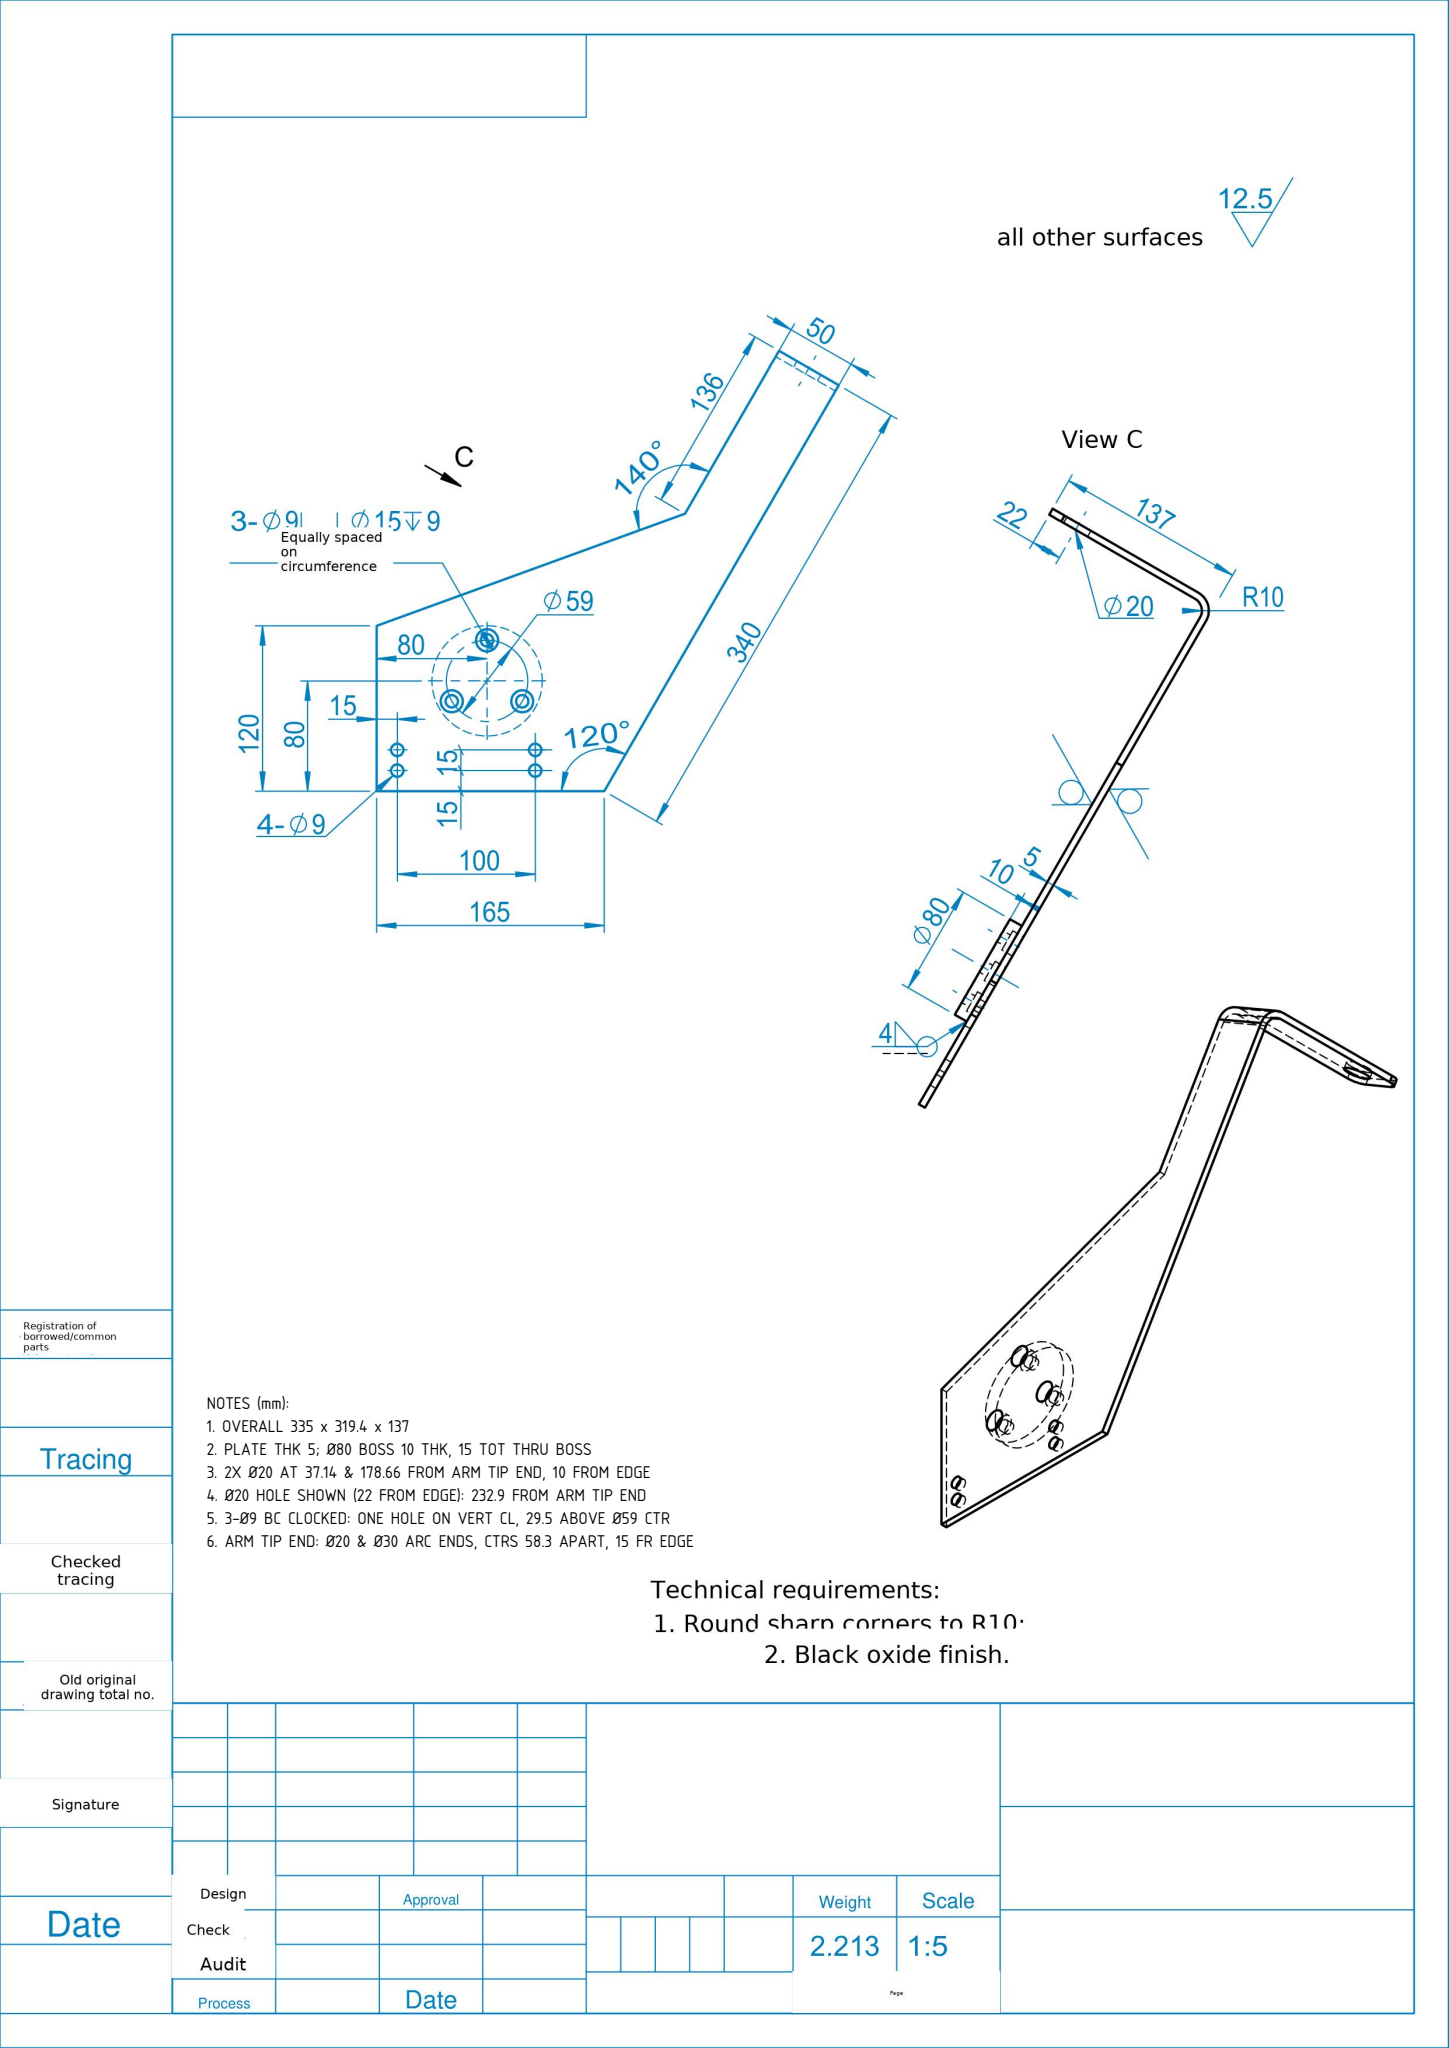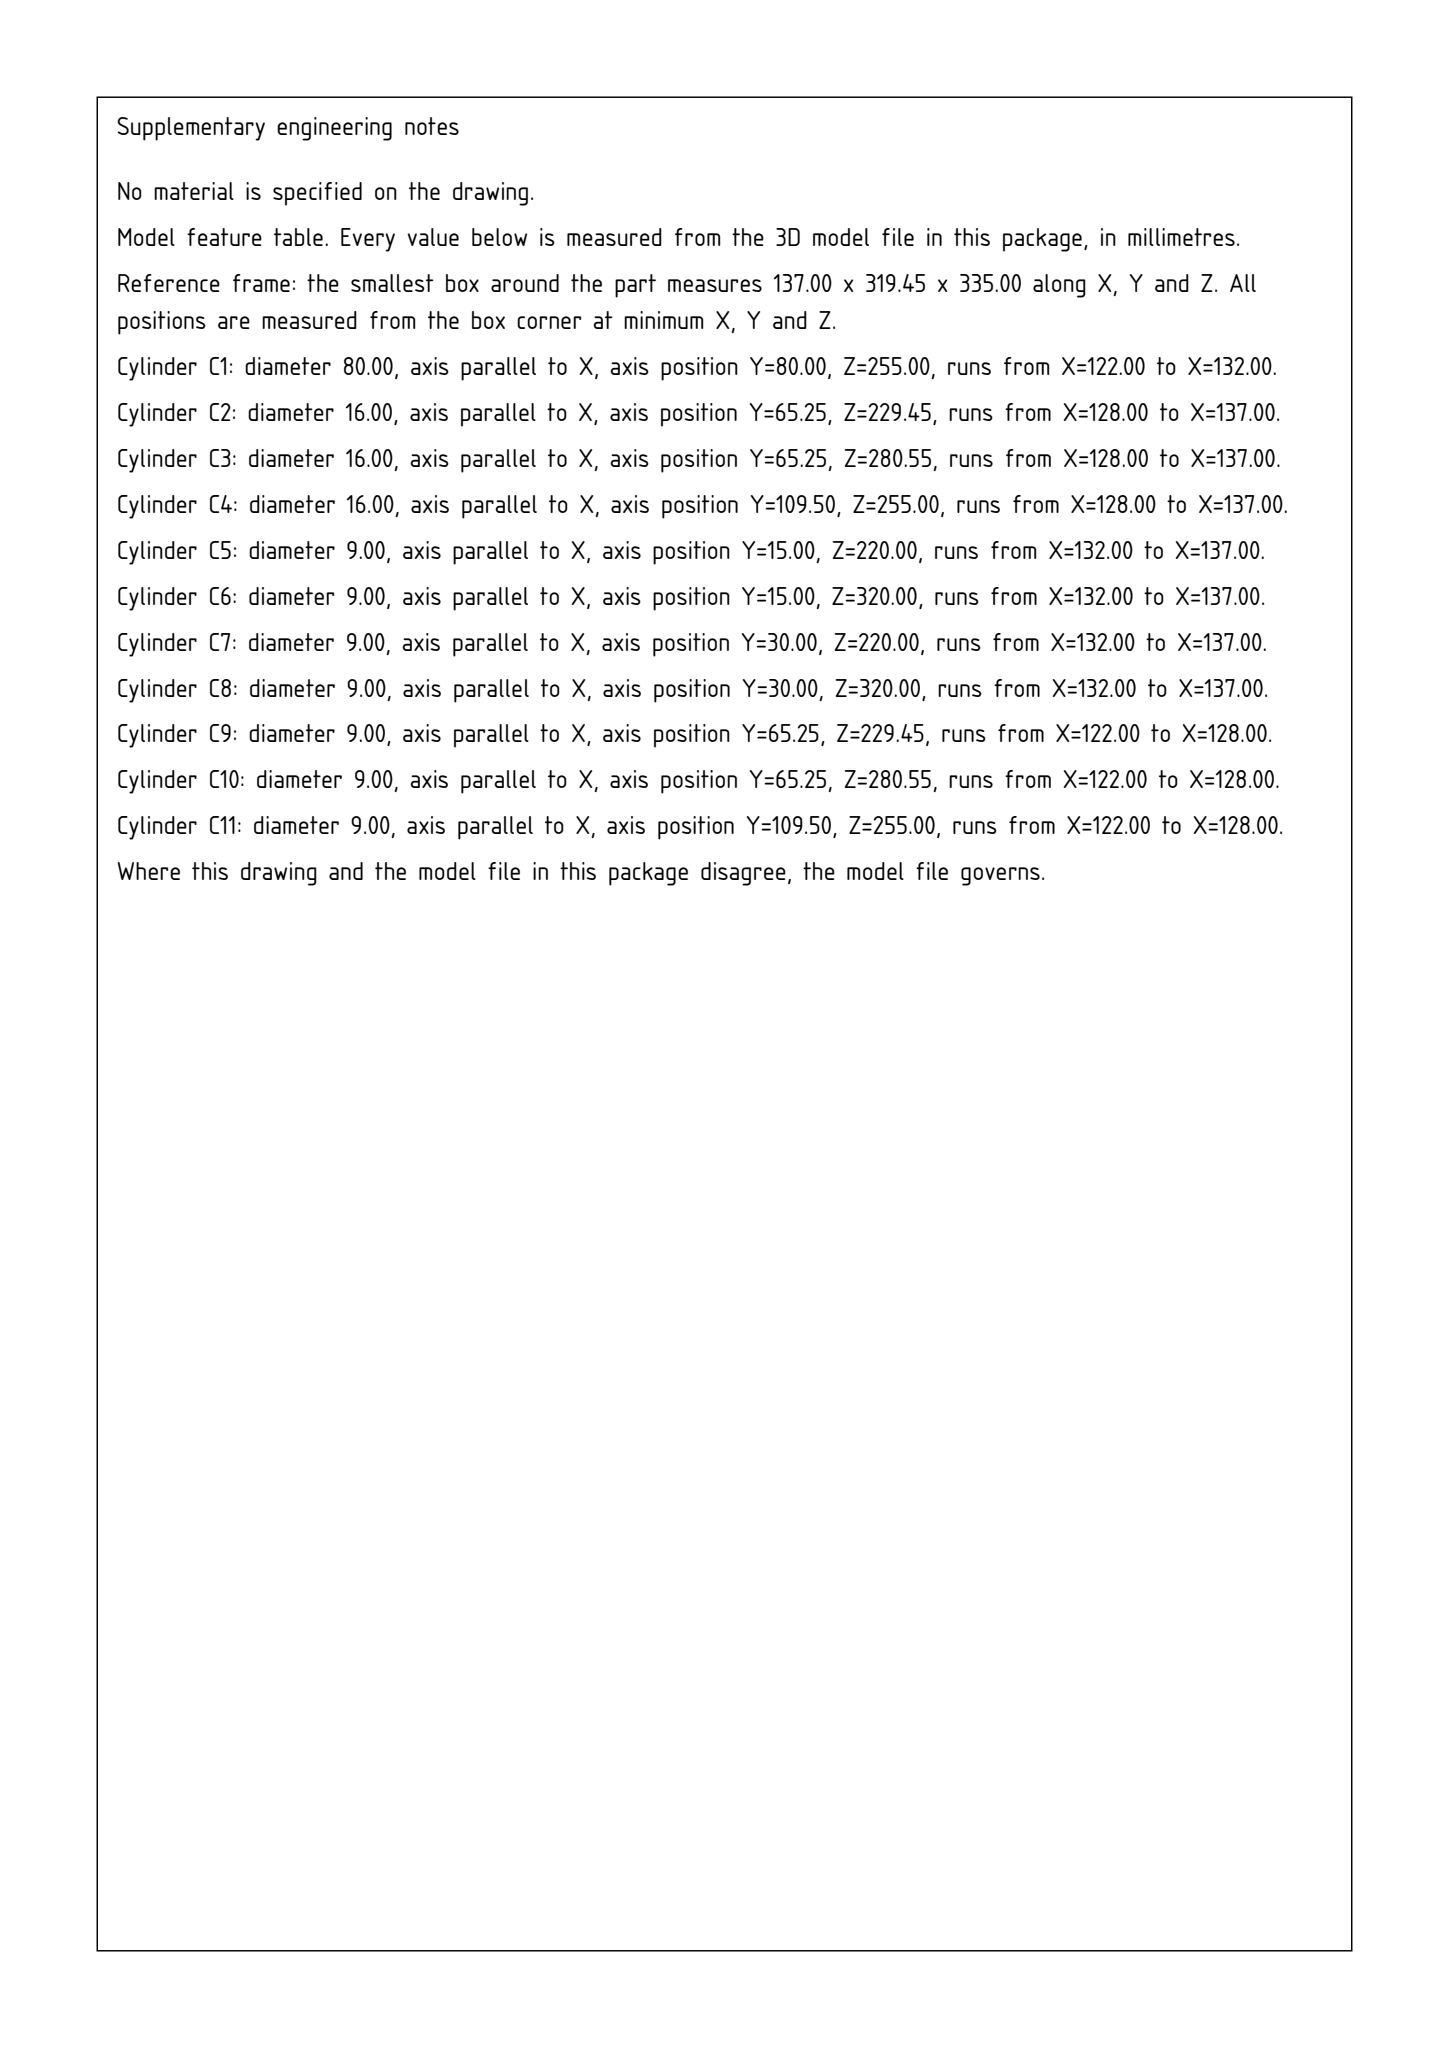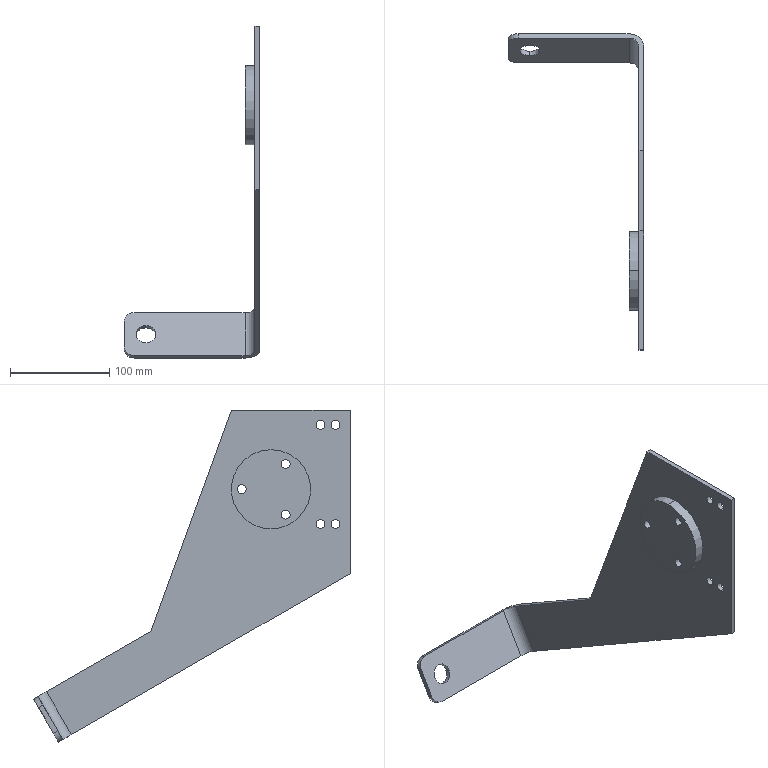Part | SolidWorks | mm | 1 solid | 42 faces | box 137 x 319.45 x 335 mm | volume 281946 mm3 | cylinder 28 | plane 14 | commonest cylinder face diameters 9 x14 16.009 x6 20 x5 80 x2 30 x1
Drawing notes:
OVERALL 335 x 319.4 x 137 | from the solid: bbox_xyz [137.0, 319.449, 335.0]
PLATE THK 5; Ø80 BOSS 10 THK, 15 TOT THRU BOSS | from the solid: x-planes 122/132/137: plate 132-137=5; Ø80 cyl len 10 (x122-132); 3-Ø9 len 6 + Ø16 CBORE DP9 = 15
2X Ø20 AT 37.14 & 178.66 FROM ARM TIP END, 10 FROM EDGE | from the solid: Ø20 cyls, axis Y, pos (x=10, z=37.14) and (x=10, z=178.66)
Ø20 HOLE SHOWN (22 FROM EDGE): 232.9 FROM ARM TIP END | from the solid: Ø20 cyl, axis Y, pos x=22.0, z=232.9 (bbox z=0 = arm tip end)
3-Ø9 BC CLOCKED: ONE HOLE ON VERT CL, 29.5 ABOVE Ø59 CTR | from the solid: Ø9 holes at (y109.5,z255),(y65.25,z229.45),(y65.25,z280.55); ctr y80 z255, R29.5, 120° spacing
ARM TIP END: Ø20 & Ø30 ARC ENDS, CTRS 58.3 APART, 15 FR EDGE | from the solid: Ø20 cyl axis Z at (x122, y281.46) & Ø30 cyl axis Z at (x122, y339.76); Δy=58.3; x=122 vs face x=137